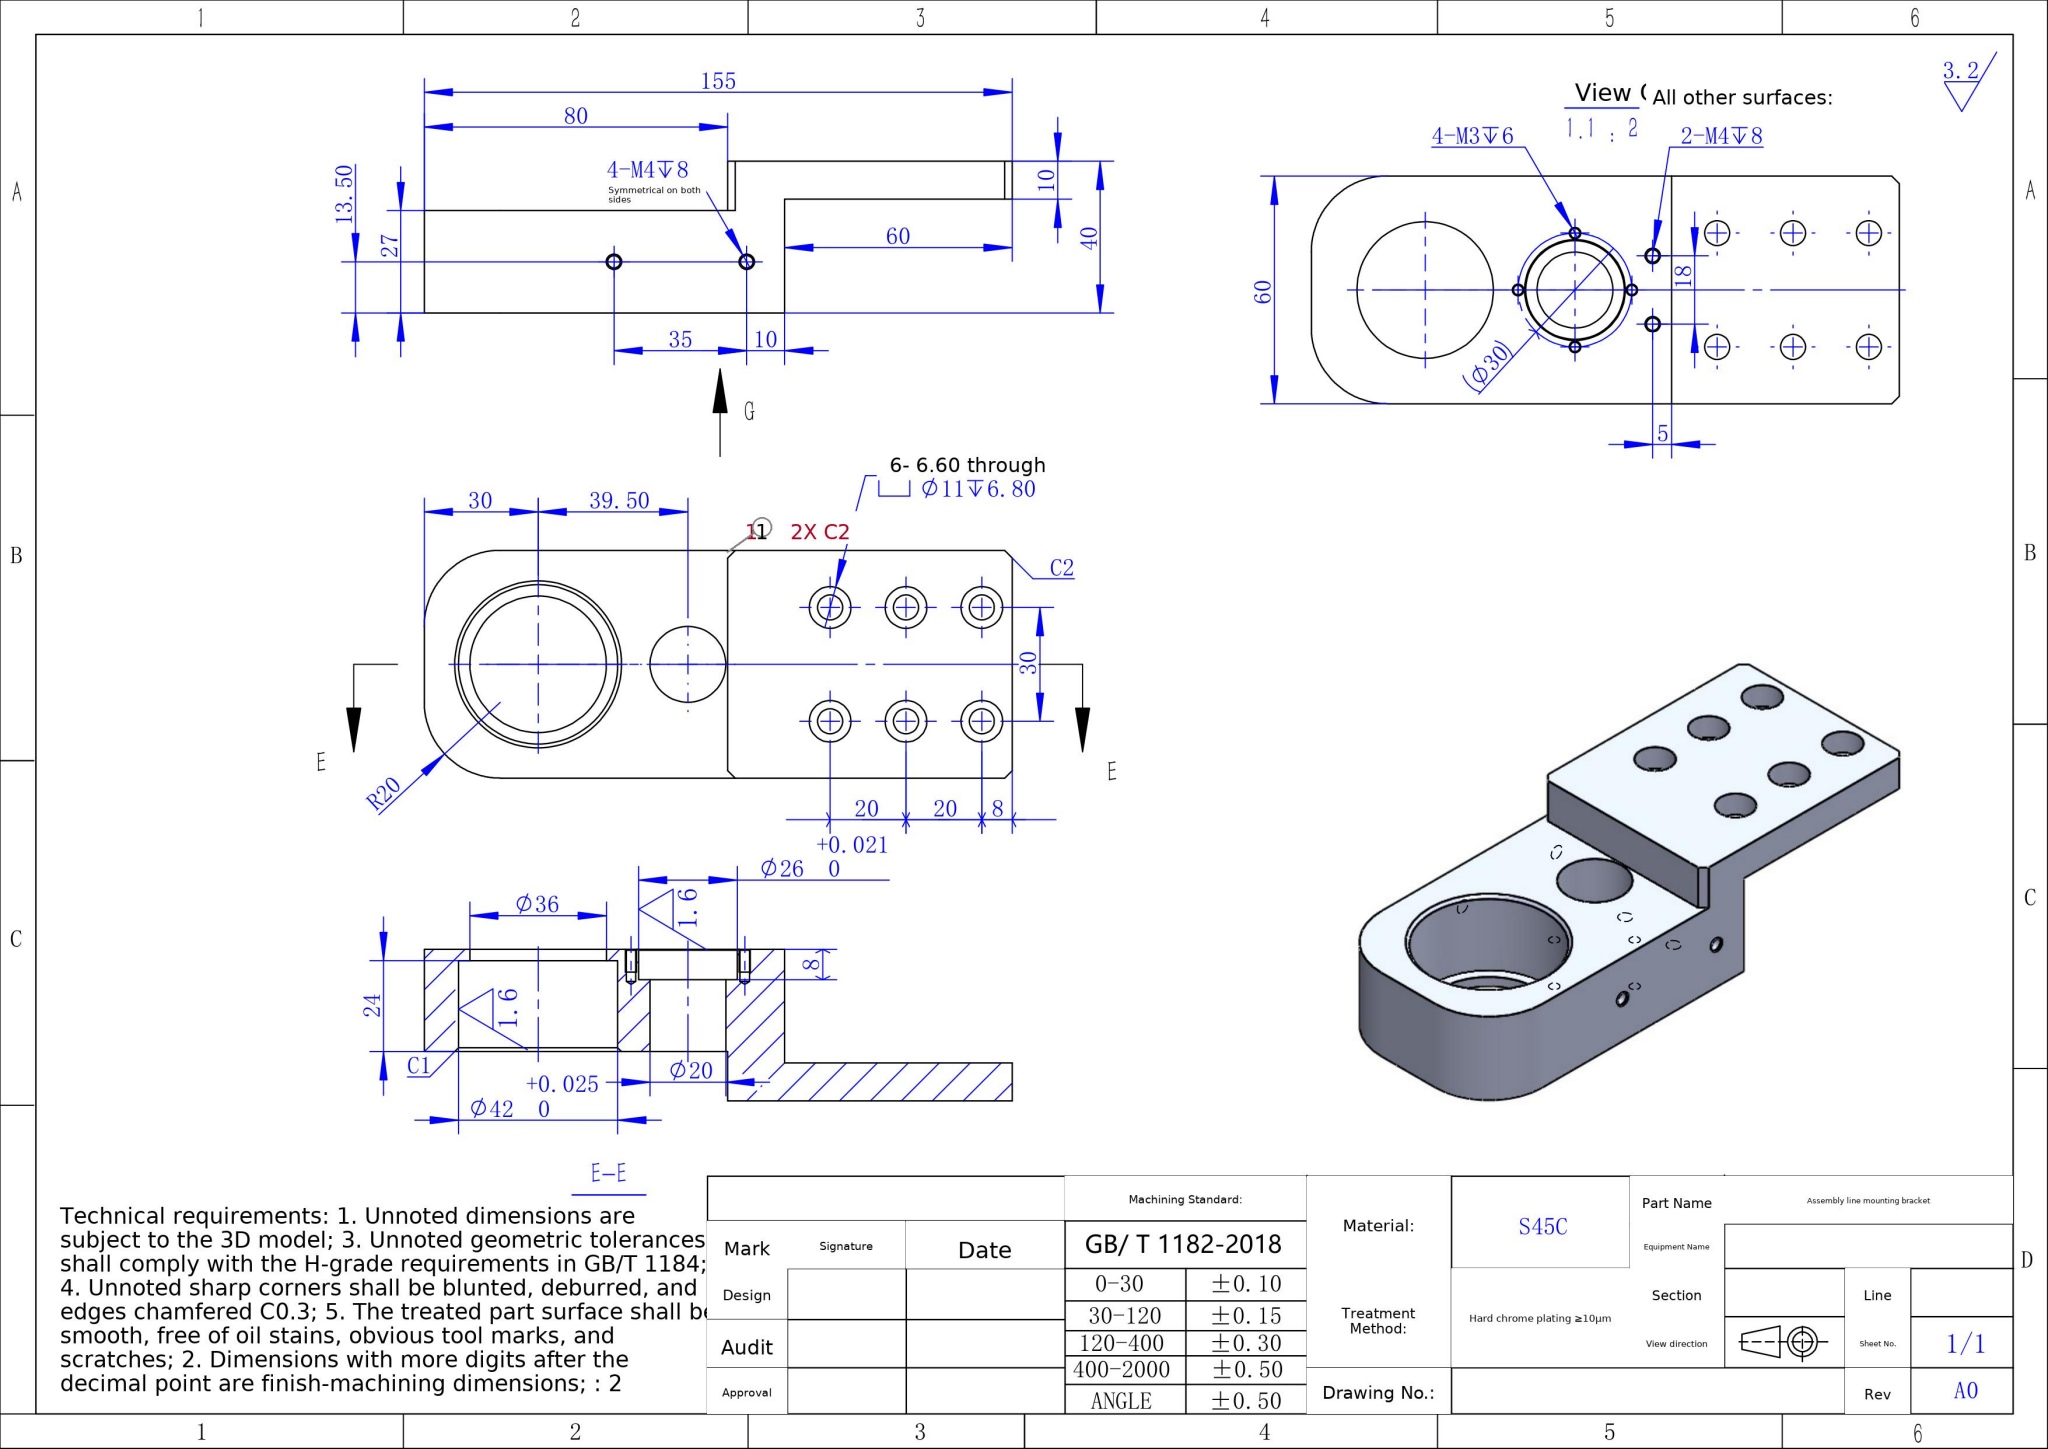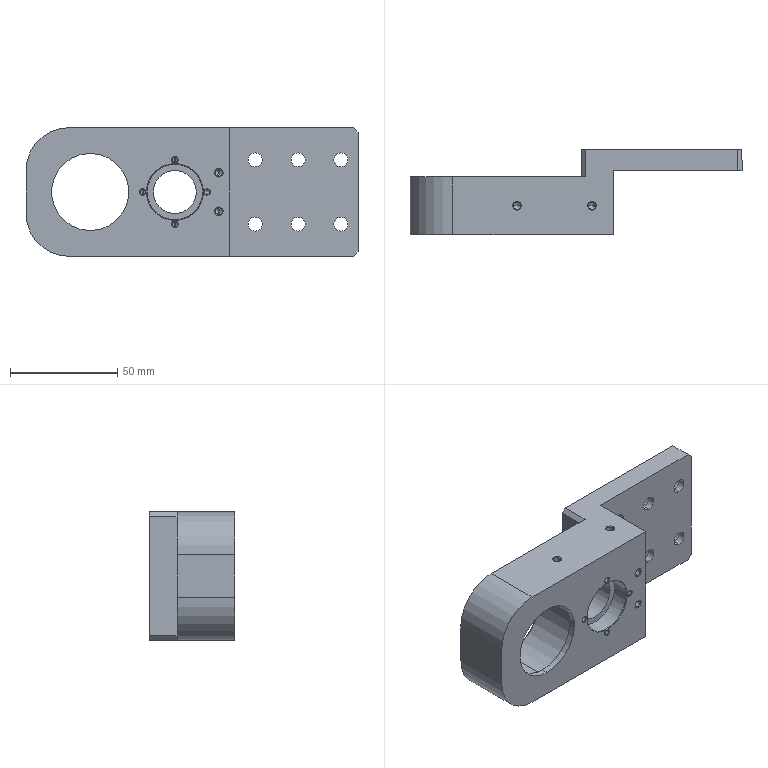Part | SolidWorks | mm | material S45C | 1 solid | 120 faces | box 155 x 40 x 60 mm | volume 144962 mm3 | cylinder 54 | cone 44 | plane 22 | commonest cylinder face diameters 3.3 x12 11 x12 6.6 x12 2.5 x8 26 x2 42 x2 36 x2 20 x2
build123d program:
from build123d import *

# Parameters (mm, degrees)
BOSS_EXTRUDE1_DEPTH         = 30
FILLET1_R                   = 20
SKETCH2_R                   = 18
CUT_EXTRUDE1_DEPTH          = 60
SKETCH3_R                   = 21
CUT_EXTRUDE2_DEPTH          = 24
CHAMFER1_SIZE               = 2
SKETCH4_R                   = 3.3
CUT_EXTRUDE3_DEPTH          = 163.865
SKETCH5_R                   = 5.5
CUT_EXTRUDE4_DEPTH          = 6.8
M4_TAPPED_HOLE2_D           = 3.3
M4_TAPPED_HOLE2_DEPTH       = 11.5
M4_TAPPED_HOLE2_CSINK_D     = 4.05
M4_TAPPED_HOLE2_CSINK_ANGLE = 90
M4_TAPPED_HOLE2_TIP         = 0.9914
SKETCH8_R                   = 10
CUT_EXTRUDE5_DEPTH          = 163.865
SKETCH9_R                   = 13
CUT_EXTRUDE6_DEPTH          = 8
M3_TAPPED_HOLE2_D           = 2.5
M3_TAPPED_HOLE2_DEPTH       = 8.5
M3_TAPPED_HOLE2_CSINK_D     = 3.05
M3_TAPPED_HOLE2_CSINK_ANGLE = 90
M3_TAPPED_HOLE2_TIP         = 0.7511
M4_TAPPED_HOLE3_AT_2_COUNT  = 2
M4_TAPPED_HOLE3_AT_2_PITCH  = 35
CHAMFER2_SIZE               = 1
CHAMFER3_SIZE               = 0.3


with BuildPart() as part:
    # Sketch1 → Boss-Extrude1 (new, symmetric)
    with BuildSketch(Plane.XY):
        Polygon((0, 0), (80, 0), (80, 13), (155, 13), (155, 3), (95, 3), (95, -27), (0, -27), align=None)
    extrude(amount=BOSS_EXTRUDE1_DEPTH, both=True)

    # Fillet1
    fillet1_edges = [part.edges().sort_by_distance(p)[0] for p in [
        (0, -13.5, -30),
        (0, -13.5, 30),
    ]]
    fillet(fillet1_edges, radius=FILLET1_R)

    # Sketch2 → Cut-Extrude1 (cut)
    with BuildSketch(Plane(origin=(0, 0, 0), x_dir=(1, 0, 0), z_dir=(0, 1, 0))):
        with Locations(Location((30, 0, 0), (0, 0, 270))):
            Circle(SKETCH2_R)
    extrude(amount=-CUT_EXTRUDE1_DEPTH, mode=Mode.SUBTRACT)

    # Sketch3 → Cut-Extrude2 (cut)
    with BuildSketch(Plane(origin=(0, 0, 0), x_dir=(1, 0, 0), z_dir=(0, 1, 0))):
        with Locations(Location((30, 0, 0), (0, 0, 270))):
            Circle(SKETCH3_R)
    extrude(amount=-CUT_EXTRUDE2_DEPTH, mode=Mode.SUBTRACT)

    # Chamfer1
    chamfer1_edges = [part.edges().sort_by_distance(p)[0] for p in [
        (155, 8, 30),
        (80, 6.5, 30),
        (80, 6.5, -30),
        (155, 8, -30),
    ]]
    chamfer(chamfer1_edges, length=CHAMFER1_SIZE)

    # Sketch4 → Cut-Extrude3 (cut, through all)
    with BuildSketch(Plane(origin=(0, 13, 0), x_dir=(1, 0, 0), z_dir=(0, 1, 0))):
        with Locations(Location((147, 15, 0), (0, 0, 270))):
            Circle(SKETCH4_R)
        with Locations(Location((127, 15, 0), (0, 0, 270))):
            Circle(SKETCH4_R)
        with Locations(Location((107, 15, 0), (0, 0, 270))):
            Circle(SKETCH4_R)
        with Locations(Location((147, -15, 0), (0, 0, 180))):
            Circle(SKETCH4_R)
        with Locations(Location((127, -15, 0), (0, 0, 180))):
            Circle(SKETCH4_R)
        with Locations(Location((107, -15, 0), (0, 0, 180))):
            Circle(SKETCH4_R)
    extrude(amount=-CUT_EXTRUDE3_DEPTH, mode=Mode.SUBTRACT)

    # Sketch5 → Cut-Extrude4 (cut)
    with BuildSketch(Plane(origin=(0, 13, 0), x_dir=(1, 0, 0), z_dir=(0, 1, 0))):
        with Locations(Location((107, 15, 0), (0, 0, 270))):
            Circle(SKETCH5_R)
        with Locations(Location((127, 15, 0), (0, 0, 270))):
            Circle(SKETCH5_R)
        with Locations(Location((147, 15, 0), (0, 0, 270))):
            Circle(SKETCH5_R)
        with Locations(Location((107, -15, 0), (0, 0, 270))):
            Circle(SKETCH5_R)
        with Locations(Location((127, -15, 0), (0, 0, 270))):
            Circle(SKETCH5_R)
        with Locations(Location((147, -15, 0), (0, 0, 270))):
            Circle(SKETCH5_R)
    extrude(amount=-CUT_EXTRUDE4_DEPTH, mode=Mode.SUBTRACT)

    # M4 Tapped Hole2
    with Locations(Plane(origin=(0, -27, 0), x_dir=(-1, 0, 0), z_dir=(0, -1, 0))):
        with Locations((-90, -9), (-90, 9)):
            CounterSinkHole(M4_TAPPED_HOLE2_D / 2, M4_TAPPED_HOLE2_CSINK_D / 2, depth=M4_TAPPED_HOLE2_DEPTH, counter_sink_angle=M4_TAPPED_HOLE2_CSINK_ANGLE)
            with Locations((0, 0, -(M4_TAPPED_HOLE2_DEPTH + M4_TAPPED_HOLE2_TIP / 2))):  # 118° drill point
                Cone(0, M4_TAPPED_HOLE2_D / 2, M4_TAPPED_HOLE2_TIP, mode=Mode.SUBTRACT)

    # Sketch8 → Cut-Extrude5 (cut, through all)
    with BuildSketch(Plane.XZ.offset(27)):
        with Locations((69.5, 0)):
            Circle(SKETCH8_R)
    extrude(amount=-CUT_EXTRUDE5_DEPTH, mode=Mode.SUBTRACT)

    # Sketch9 → Cut-Extrude6 (cut)
    with BuildSketch(Plane.XZ.offset(27)):
        with Locations((69.5, 0)):
            Circle(SKETCH9_R)
    extrude(amount=-CUT_EXTRUDE6_DEPTH, mode=Mode.SUBTRACT)

    # M3 Tapped Hole2
    with Locations(Plane(origin=(0, -27, 0), x_dir=(-1, 0, 0), z_dir=(0, -1, 0))):
        with Locations((-69.5, 15), (-54.5, 0), (-84.5, 0), (-69.5, -15)):
            CounterSinkHole(M3_TAPPED_HOLE2_D / 2, M3_TAPPED_HOLE2_CSINK_D / 2, depth=M3_TAPPED_HOLE2_DEPTH, counter_sink_angle=M3_TAPPED_HOLE2_CSINK_ANGLE)
            with Locations((0, 0, -(M3_TAPPED_HOLE2_DEPTH + M3_TAPPED_HOLE2_TIP / 2))):  # 118° drill point
                Cone(0, M3_TAPPED_HOLE2_D / 2, M3_TAPPED_HOLE2_TIP, mode=Mode.SUBTRACT)

    # Sketch13 → M4 Tapped Hole3 (revolve, cut)
    with BuildSketch(Plane(origin=(85, -13.5, 30), x_dir=(0, -1, 0), z_dir=(1, 0, 0))):
        Polygon((0, 0), (0, 12.491), (1.65, 11.5), (1.65, 0.375), (2.025, 0), align=None)
    m4_tapped_hole3 = revolve(axis=Axis((85, -13.5, 36.35), (0, 0, -1)), mode=Mode.SUBTRACT)

    # M4 Tapped Hole3 at 2: M4 Tapped Hole3 ×2
    with Locations(*[(-i * M4_TAPPED_HOLE3_AT_2_PITCH, 0, 0) for i in range(1, M4_TAPPED_HOLE3_AT_2_COUNT)]):
        add(m4_tapped_hole3, mode=Mode.SUBTRACT)

    # Mirror1: M4 Tapped Hole3 across plane
    add(m4_tapped_hole3.mirror(Plane.XY), mode=Mode.SUBTRACT)

    # Mirror1 copy 1 sketch → Mirror1 copy 1 (revolve, cut)
    with BuildSketch(Plane(origin=(50, -13.5, -30), x_dir=(0, -1, 0), z_dir=(1, 0, 0))):
        Polygon((0, 0), (0, -12.491), (1.65, -11.5), (1.65, -0.375), (2.025, 0), align=None)
    revolve(axis=Axis((50, -13.5, -36.35), (0, 0, -1)), mode=Mode.SUBTRACT)

    # Chamfer2
    chamfer2_edges = [part.edges().sort_by_distance(p)[0] for p in [
        (30, 0, -21),
    ]]
    chamfer(chamfer2_edges, length=CHAMFER2_SIZE)

    # Chamfer3
    chamfer3_edges = [part.edges().sort_by_distance(p)[0] for p in [
        (56.5, -27, 0),
    ]]
    chamfer(chamfer3_edges, length=CHAMFER3_SIZE)


solid = part.part